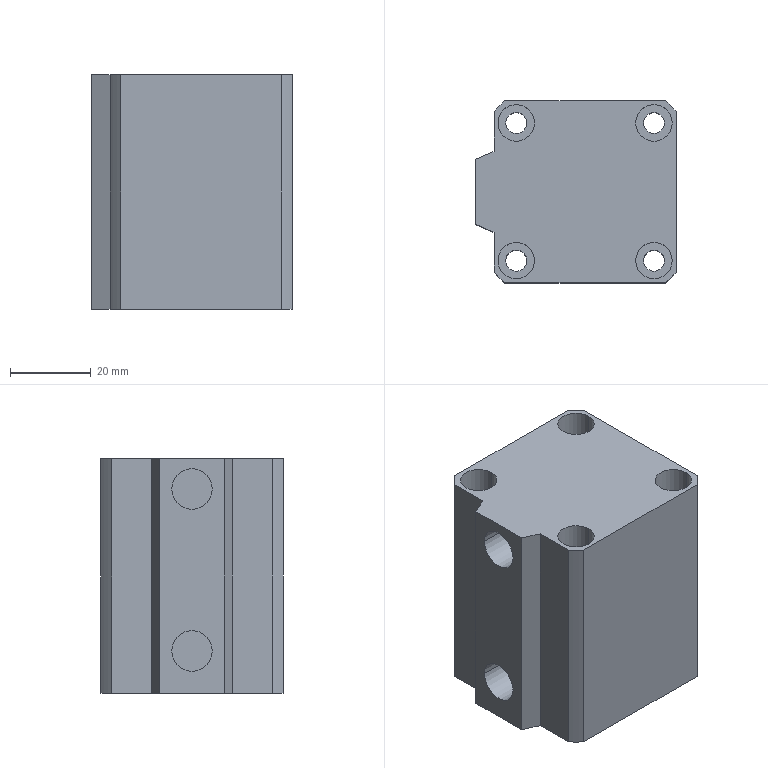Component | SolidWorks | ACQS-32X25CylinderBody-2 | 1 solid | 55 faces | box 49.5 x 45 x 58 mm | volume 105826 mm3 | cylinder 34 | plane 21 | commonest cylinder face diameters 9 x16 5.2 x8 10 x4 60 x4 16 x2
build123d program:
from build123d import *

# Parameters (mm, degrees)
SKETCH1_W          = 45
SKETCH1_H          = 45
EXTRUDE1_DEPTH     = 58
SKETCH2_OUTSIDE_W  = 64.22
SKETCH2_OUTSIDE_H  = 64.22
SKETCH2_OUTSIDE_R  = 30
CUT_EXTRUDE1_DEPTH = 87.105
SKETCH3_2_R        = 4.5
CUT_EXTRUDE2_DEPTH = 7
SKETCH4_R          = 2.6
CUT_EXTRUDE3_DEPTH = 87.105
CUT_EXTRUDE4_START = -58
SKETCH3_2_2_R      = 4.5
CUT_EXTRUDE4_DEPTH = 7
EXTRUDE2_DEPTH     = 58
SKETCH6_R          = 8
CUT_EXTRUDE5_DEPTH = 35.5
SKETCH7_R          = 5
CUT_EXTRUDE6_DEPTH = 7


with BuildPart() as part:
    # Sketch1 → Extrude1 (new body)
    with BuildSketch(Plane(origin=(0, 0, 0), x_dir=(1, 0, 0), z_dir=(0, 1, 0))):
        with Locations((22.5, -22.5)):
            Rectangle(SKETCH1_W, SKETCH1_H)
    extrude(amount=EXTRUDE1_DEPTH)

    # Sketch2 outside → Cut-Extrude1 (cut, through all)
    with BuildSketch(Plane(origin=(0, 58, 0), x_dir=(1, 0, 0), z_dir=(0, 1, 0))):
        with Locations((22.5, -22.5)):
            Rectangle(SKETCH2_OUTSIDE_W, SKETCH2_OUTSIDE_H)
        with Locations((22.5, -22.5)):
            Circle(SKETCH2_OUTSIDE_R, mode=Mode.SUBTRACT)
    extrude(amount=-CUT_EXTRUDE1_DEPTH, mode=Mode.SUBTRACT)

    # Sketch3_2 → Cut-Extrude2 (cut)
    with BuildSketch(Plane(origin=(0, 58, 0), x_dir=(1, 0, 0), z_dir=(0, 1, 0))):
        with Locations(Location((5.5, -5.5, 0), (0, 0, 270))):
            Circle(SKETCH3_2_R)
        with Locations(Location((39.5, -5.5, 0), (0, 0, 270))):
            Circle(SKETCH3_2_R)
        with Locations(Location((39.5, -39.5, 0), (0, 0, 270))):
            Circle(SKETCH3_2_R)
        with Locations(Location((5.5, -39.5, 0), (0, 0, 270))):
            Circle(SKETCH3_2_R)
    extrude(amount=-CUT_EXTRUDE2_DEPTH, mode=Mode.SUBTRACT)

    # Sketch4 → Cut-Extrude3 (cut, through all)
    with BuildSketch(Plane(origin=(0, 58, 0), x_dir=(1, 0, 0), z_dir=(0, 1, 0))):
        with Locations(Location((5.5, -5.5, 0), (0, 0, 270))):
            Circle(SKETCH4_R)
        with Locations(Location((39.5, -5.5, 0), (0, 0, 270))):
            Circle(SKETCH4_R)
        with Locations(Location((39.5, -39.5, 0), (0, 0, 270))):
            Circle(SKETCH4_R)
        with Locations(Location((5.5, -39.5, 0), (0, 0, 270))):
            Circle(SKETCH4_R)
    extrude(amount=-CUT_EXTRUDE3_DEPTH, mode=Mode.SUBTRACT)

    # Sketch3_2 2 → Cut-Extrude4 (cut)
    with BuildSketch(Plane(origin=(0, 58, 0), x_dir=(1, 0, 0), z_dir=(0, 1, 0)).offset(CUT_EXTRUDE4_START)):
        with Locations(Location((5.5, -5.5, 0), (0, 0, 270))):
            Circle(SKETCH3_2_2_R)
        with Locations(Location((39.5, -5.5, 0), (0, 0, 270))):
            Circle(SKETCH3_2_2_R)
        with Locations(Location((39.5, -39.5, 0), (0, 0, 270))):
            Circle(SKETCH3_2_2_R)
        with Locations(Location((5.5, -39.5, 0), (0, 0, 270))):
            Circle(SKETCH3_2_2_R)
    extrude(amount=CUT_EXTRUDE4_DEPTH, mode=Mode.SUBTRACT)

    # Sketch5 → Extrude2 (add)
    with BuildSketch(Plane(origin=(0, 58, 0), x_dir=(1, 0, 0), z_dir=(0, 1, 0))):
        Polygon((12.5, 0), (14.5, 4.5), (30.5, 4.5), (32.5, 0), align=None)
    extrude(amount=-EXTRUDE2_DEPTH)

    # Sketch6 → Cut-Extrude5 (cut)
    with BuildSketch(Plane(origin=(0, 58, 0), x_dir=(1, 0, 0), z_dir=(0, 1, 0))):
        with Locations(Location((22.5, -22.5, 0), (0, 0, 270))):
            Circle(SKETCH6_R)
    extrude(amount=-CUT_EXTRUDE5_DEPTH, mode=Mode.SUBTRACT)

    # Sketch7 → Cut-Extrude6 (cut)
    with BuildSketch(Plane(origin=(0, 0, -4.5), x_dir=(-1, 0, 0), z_dir=(0, 0, -1))):
        with Locations((-22.5, 47.5)):
            Circle(SKETCH7_R)
        with Locations((-22.5, 7.5)):
            Circle(SKETCH7_R)
    extrude(amount=-CUT_EXTRUDE6_DEPTH, mode=Mode.SUBTRACT)


solid = part.part

# Placed as in the assembly
solid = solid.moved(Location((-34.083, 68.372, -13.387), (-90, 90, 0)))